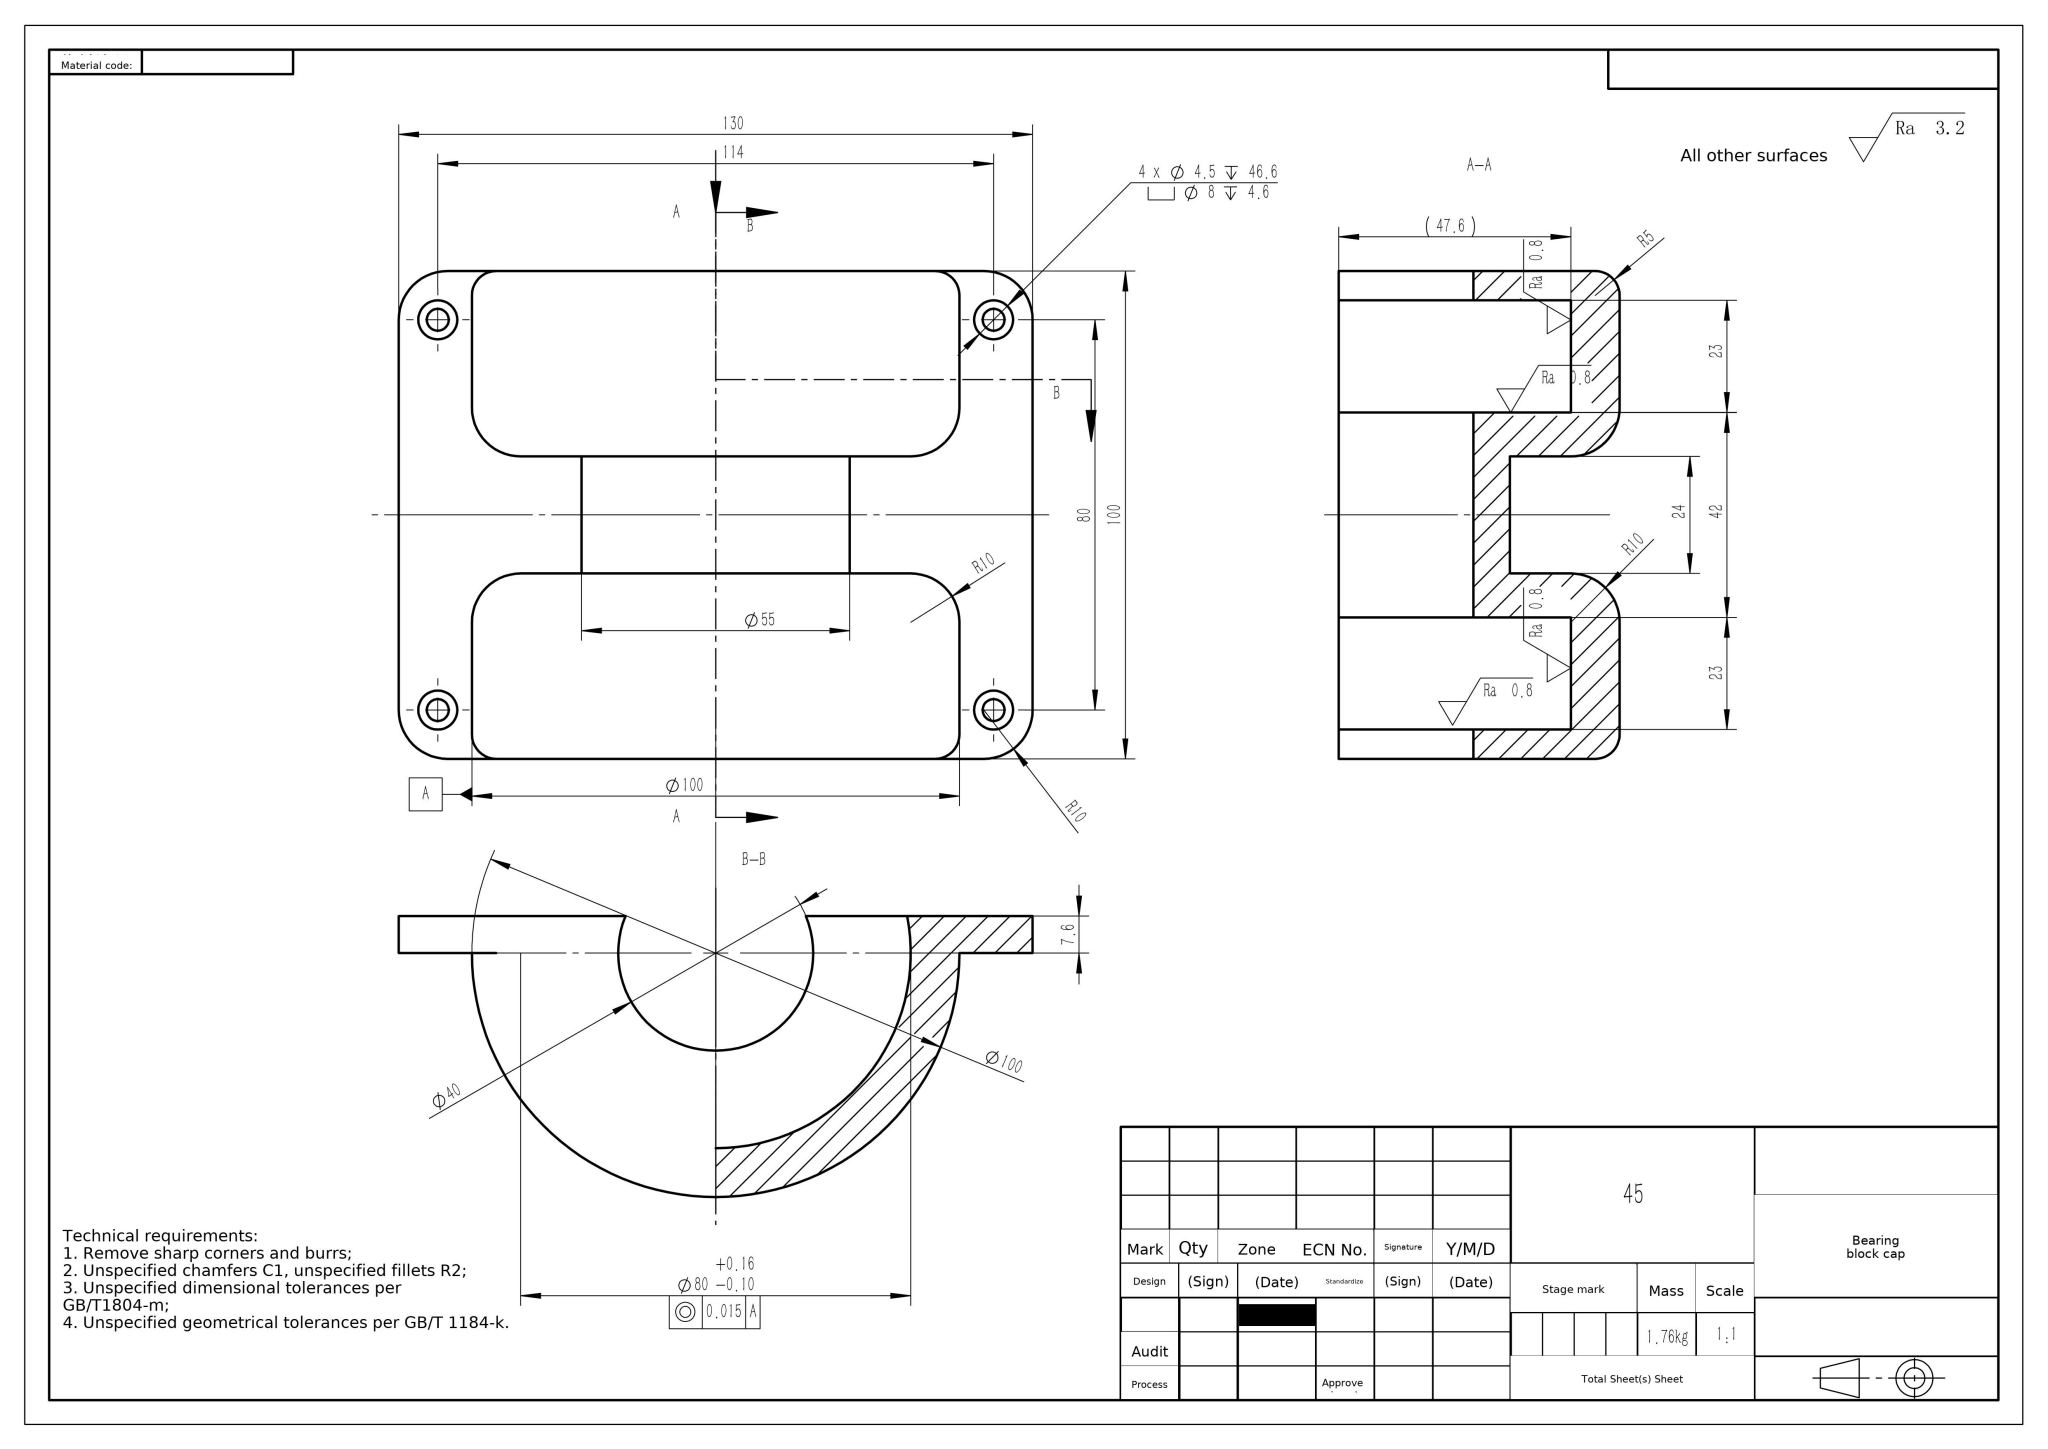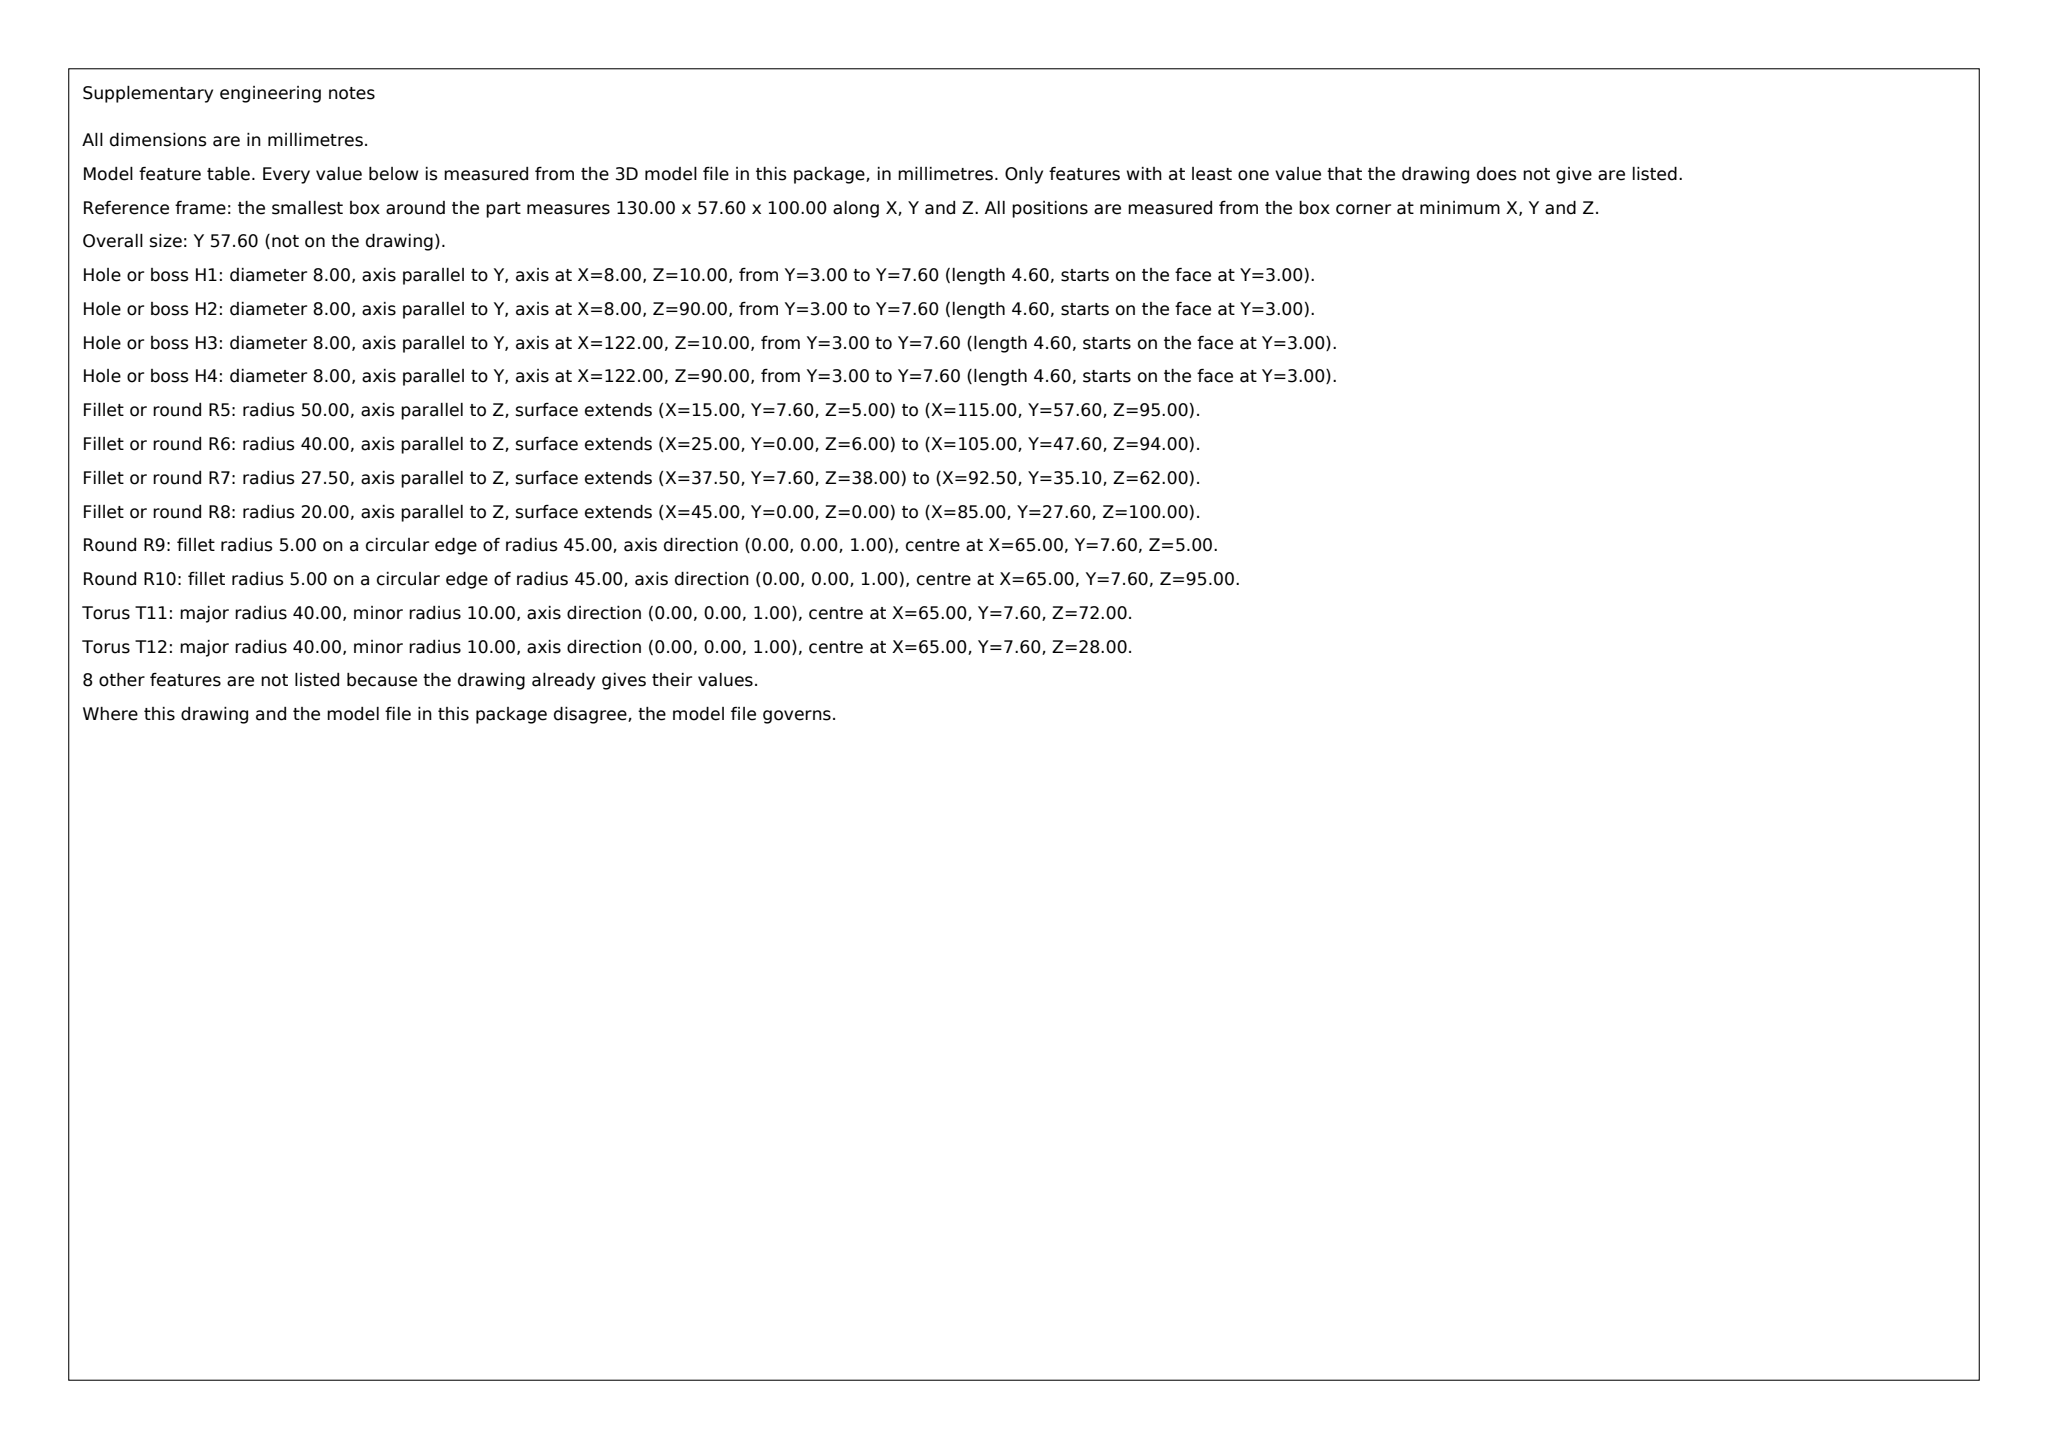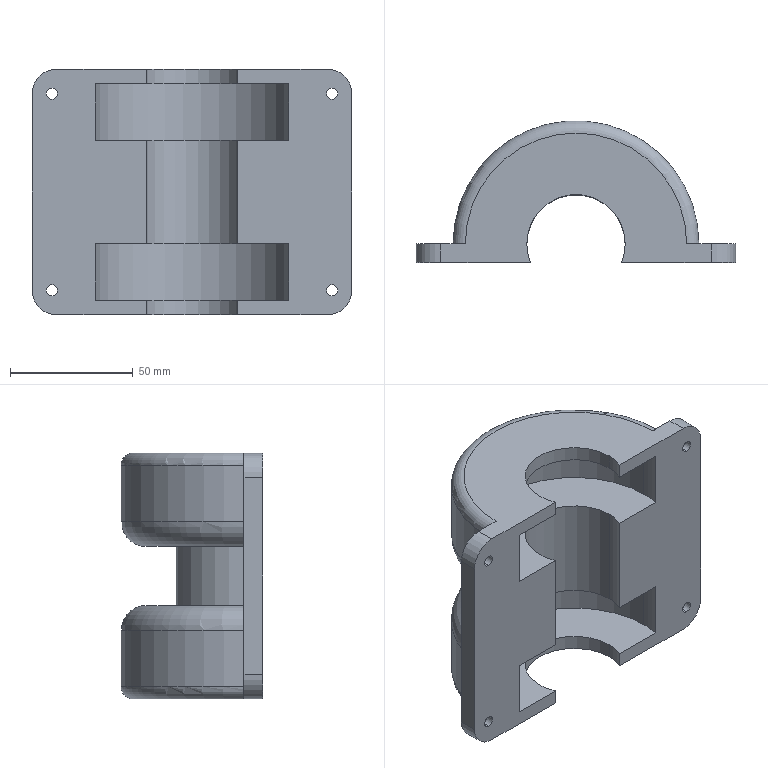Part | SolidWorks | mm | material 45 | 1 solid | 60 faces | box 130 x 57.6 x 100 mm | volume 222590 mm3 | cylinder 38 | plane 18 | torus 4 | commonest cylinder face diameters 40 x9 8 x8 4.5 x8 80 x6 20 x4 100 x2 55 x1